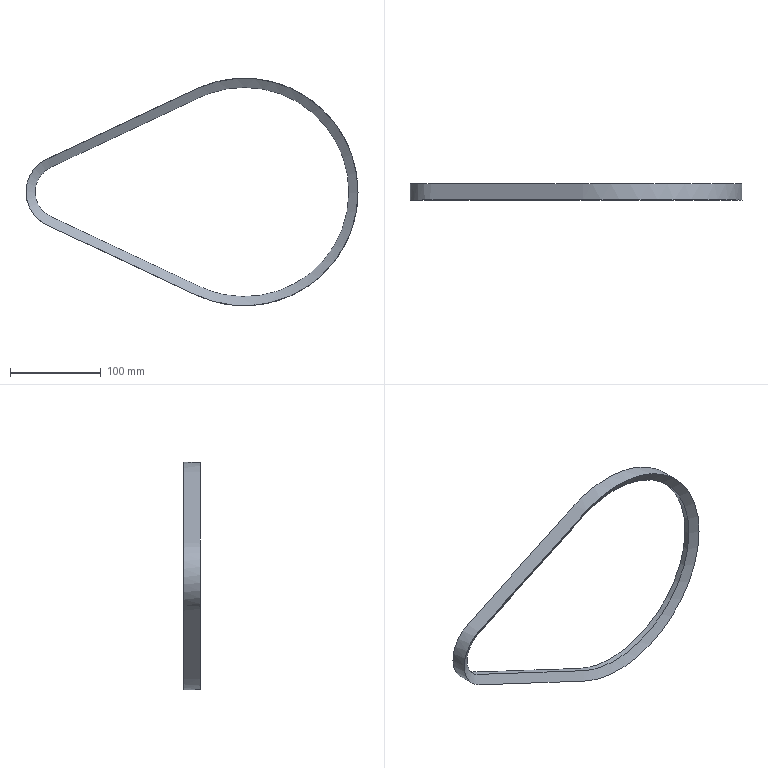Component | NX | BELT_2 | 1 solid | 4 faces | volume 111871 mm3 | spline 4